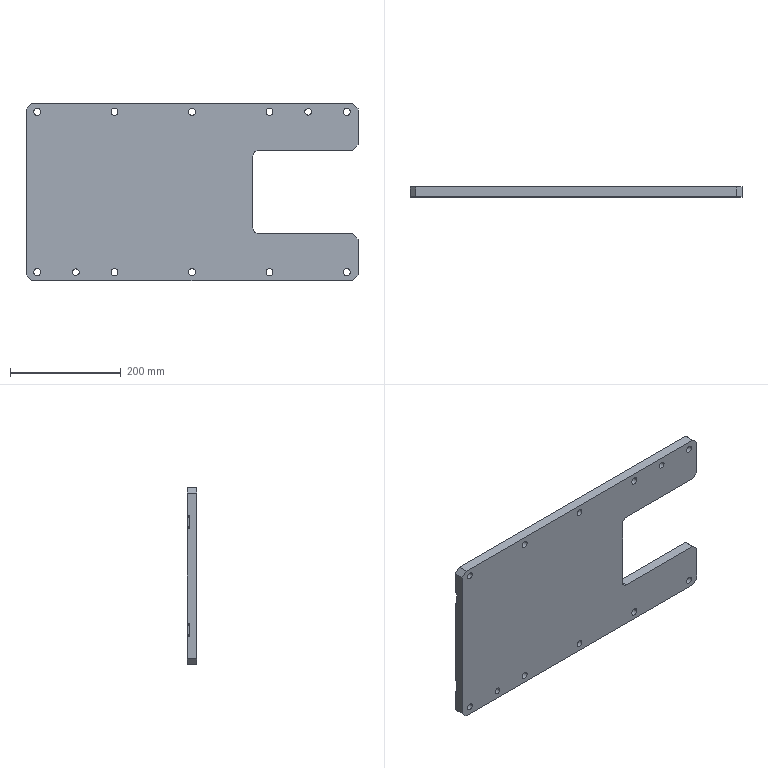Component | SolidWorks | 100-01-1 | 1 solid | 58 faces | box 600 x 18 x 320 mm | volume 2796129 mm3 | cylinder 34 | plane 24 | commonest cylinder face diameters 12.5 x20 6 x8 12 x4 20 x2 | material 45
build123d program:
from build123d import *

# Parameters (mm, degrees)
SKETCH1_W                    = 320
SKETCH1_H                    = 600
BOSS_EXTRUDE1_DEPTH          = 18
F_12_5_12_5_DIAMETER_HOLE1_D = 12.5
SKETCH4_R                    = 6
CUT_EXTRUDE1_DEPTH           = 341.476
SKETCH5_W                    = 25
SKETCH5_H                    = 580
CUT_EXTRUDE2_DEPTH           = 4
SKETCH6_R                    = 3
CUT_EXTRUDE3_DEPTH           = 4
SKETCH7_W                    = 150
SKETCH7_H                    = 190
CUT_EXTRUDE4_DEPTH           = 341.476
FILLET1_R                    = 10
CHAMFER1_SIZE                = 10


with BuildPart() as part:
    # Sketch1 → Boss-Extrude1 (new body)
    with BuildSketch(Plane(origin=(0, 0, 0), x_dir=(1, 0, 0), z_dir=(0, 1, 0))):
        Rectangle(SKETCH1_W, SKETCH1_H)
    extrude(amount=BOSS_EXTRUDE1_DEPTH)

    # 12.5 _12.5_ Diameter Hole1 (through all)
    with Locations(Plane(origin=(0, 18, 0), x_dir=(1, 0, 0), z_dir=(0, 1, 0))):
        with Locations((-145, 280), (-145, 140), (-145, 0), (-145, -140), (-145, -280)):
            f_12_5_12_5_diameter_hole1 = Hole(F_12_5_12_5_DIAMETER_HOLE1_D / 2)

    # Mirror1: 12.5 _12.5_ Diameter Hole1 across plane
    add(f_12_5_12_5_diameter_hole1.mirror(Plane(origin=(0, 0, 0), x_dir=(0, 0, 1), z_dir=(1, 0, 0))), mode=Mode.SUBTRACT)

    # Sketch4 → Cut-Extrude1 (cut, through all)
    with BuildSketch(Plane(origin=(0, 18, 0), x_dir=(1, 0, 0), z_dir=(0, 1, 0))):
        with Locations(Location((145, 210, 0), (0, 0, 270))):
            Circle(SKETCH4_R)
        with Locations(Location((-145, -210, 0), (0, 0, 270))):
            Circle(SKETCH4_R)
    extrude(amount=-CUT_EXTRUDE1_DEPTH, mode=Mode.SUBTRACT)

    # Sketch5 → Cut-Extrude2 (cut)
    with BuildSketch(Plane(origin=(0, 18, 0), x_dir=(1, 0, 0), z_dir=(0, 1, 0))):
        with Locations((97.5, 10)):
            Rectangle(SKETCH5_W, SKETCH5_H)
    cut_extrude2 = extrude(amount=-CUT_EXTRUDE2_DEPTH, mode=Mode.SUBTRACT)

    # Sketch6 → Cut-Extrude3 (cut)
    with BuildSketch(Plane(origin=(0, 18, 0), x_dir=(1, 0, 0), z_dir=(0, 1, 0))):
        with Locations((107.88, -277.88)):
            Circle(SKETCH6_R)
        with Locations((87.12, -277.88)):
            Circle(SKETCH6_R)
    cut_extrude3 = extrude(amount=-CUT_EXTRUDE3_DEPTH, mode=Mode.SUBTRACT)

    # Mirror2: Cut-Extrude2, Cut-Extrude3 across plane
    add(cut_extrude2.mirror(Plane(origin=(0, 0, 0), x_dir=(0, 0, 1), z_dir=(1, 0, 0))), mode=Mode.SUBTRACT)
    add(cut_extrude3.mirror(Plane(origin=(0, 0, 0), x_dir=(0, 0, 1), z_dir=(1, 0, 0))), mode=Mode.SUBTRACT)

    # Sketch7 → Cut-Extrude4 (cut, through all)
    with BuildSketch(Plane(origin=(0, 18, 0), x_dir=(1, 0, 0), z_dir=(0, 1, 0))):
        with Locations((0, -205)):
            Rectangle(SKETCH7_W, SKETCH7_H)
    extrude(amount=-CUT_EXTRUDE4_DEPTH, mode=Mode.SUBTRACT)

    # Fillet1
    fillet1_edges = [part.edges().sort_by_distance(p)[0] for p in [
        (75, 9, 110),
        (-75, 9, 110),
    ]]
    fillet(fillet1_edges, radius=FILLET1_R)

    # Chamfer1
    chamfer1_edges = [part.edges().sort_by_distance(p)[0] for p in [
        (75, 9, 300),
        (-75, 9, 300),
        (-160, 9, -300),
        (160, 9, -300),
        (160, 9, 300),
        (-160, 9, 300),
    ]]
    chamfer(chamfer1_edges, length=CHAMFER1_SIZE)


solid = part.part

# Placed as in the assembly
solid = solid.moved(Location((0, 0, 0), (0, 90, 0)))